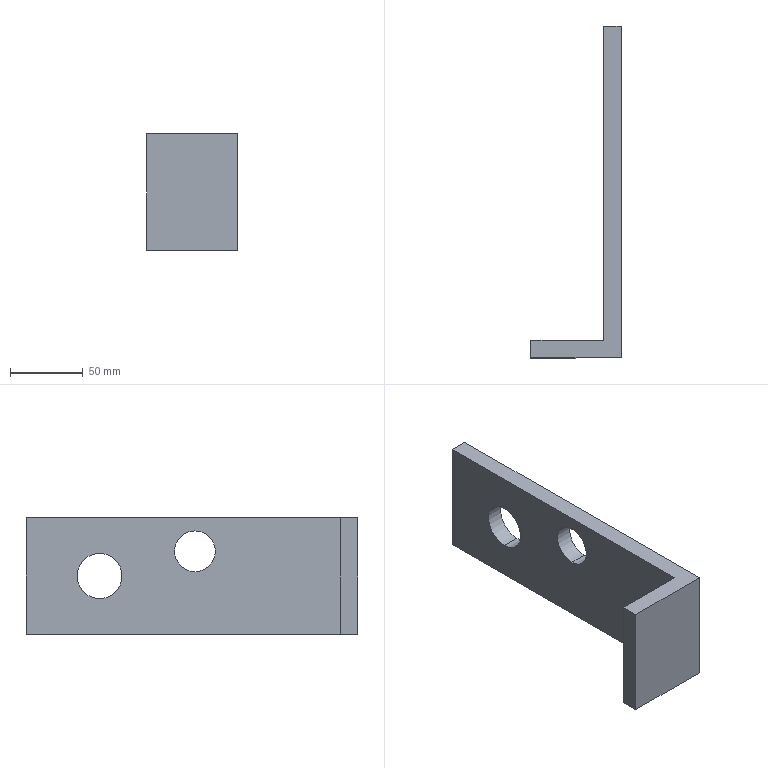Component | SolidWorks | HZ022-A001-E003-1 | 1 solid | 12 faces | box 62 x 228 x 80 mm | volume 250434 mm3 | plane 8 | cylinder 4 | commonest cylinder face diameters 28 x2 31 x2 | material AL6061
build123d program:
from build123d import *

# Parameters (mm, degrees)
SKETCH1_W           = 228
SKETCH1_H           = 80
BOSS_EXTRUDE1_DEPTH = 12
SKETCH2_W           = 80
SKETCH2_H           = 50
BOSS_EXTRUDE2_DEPTH = 12
CUT_EXTRUDE1_REACH  = 132.752
SKETCH5_R           = 15.5
SKETCH6_R           = 14
CUT_EXTRUDE2_DEPTH  = 131.752


with BuildPart() as part:
    # Sketch1 → Boss-Extrude1 (new body)
    with BuildSketch(Plane(origin=(0, 0, 0), x_dir=(1, 0, 0), z_dir=(0, 1, 0))):
        Rectangle(SKETCH1_W, SKETCH1_H)
    extrude(amount=BOSS_EXTRUDE1_DEPTH)

    # Sketch2 → Boss-Extrude2 (add)
    with BuildSketch(Plane.ZY.offset(114)):
        with Locations((0, 37)):
            Rectangle(SKETCH2_W, SKETCH2_H)
    extrude(amount=-BOSS_EXTRUDE2_DEPTH)

    # Sketch5 → Cut-Extrude1 (cut, up to next)
    with BuildSketch(Plane(origin=(0, 12, 0), x_dir=(1, 0, 0), z_dir=(0, 1, 0)), mode=Mode.PRIVATE) as cut_extrude1_sk1:
        with Locations(Location((63.5, 0, 0), (0, 0, 270))):
            Circle(SKETCH5_R)
    cut_extrude1_tool1 = extrude(cut_extrude1_sk1.sketch, amount=-CUT_EXTRUDE1_REACH, mode=Mode.PRIVATE) & part.part
    add(cut_extrude1_tool1.solids().sort_by_distance((63.5, 12, 0))[0], mode=Mode.SUBTRACT)

    # Sketch6 → Cut-Extrude2 (cut, through all)
    with BuildSketch(Plane(origin=(0, 12, 0), x_dir=(1, 0, 0), z_dir=(0, 1, 0))):
        with Locations(Location((-2, -17, 0), (0, 0, 270))):
            Circle(SKETCH6_R)
    extrude(amount=-CUT_EXTRUDE2_DEPTH, mode=Mode.SUBTRACT)


solid = part.part

# Placed as in the assembly
solid = solid.moved(Location((-77.556, 128.652, 910), (0, 0, 90)))
STEP:
#1=COLOUR_RGB('',0.7922,0.8196,0.9333);
#2=FILL_AREA_STYLE_COLOUR('',#1);
#3=FILL_AREA_STYLE('',(#2));
#4=SURFACE_STYLE_FILL_AREA(#3);
#5=SURFACE_SIDE_STYLE('',(#4));
#6=SURFACE_STYLE_USAGE(.BOTH.,#5);
#7=PRESENTATION_STYLE_ASSIGNMENT((#6));
#8=CARTESIAN_POINT('',(-3.053,4.986,35.945));
#9=VERTEX_POINT('',#8);
#10=CARTESIAN_POINT('',(-3.053,4.986,37.047));
#11=VERTEX_POINT('',#10);
#12=CARTESIAN_POINT('',(-3.053,4.986,36.496));
#13=DIRECTION('',(-1.,-0.,0.));
#14=DIRECTION('',(0.,0.,1.));
#15=AXIS2_PLACEMENT_3D('',#12,#13,#14);
#16=CIRCLE('',#15,0.5512);
#17=EDGE_CURVE('',#9,#11,#16,.T.);
#18=ORIENTED_EDGE('',*,*,#17,.F.);
#19=CARTESIAN_POINT('',(-3.526,4.986,35.945));
#20=VERTEX_POINT('',#19);
#21=CARTESIAN_POINT('',(-3.053,4.986,35.945));
#22=DIRECTION('',(-1.,-0.,0.));
#23=VECTOR('',#22,39.37);
#24=LINE('',#21,#23);
#25=EDGE_CURVE('',#9,#20,#24,.T.);
#26=ORIENTED_EDGE('',*,*,#25,.T.);
#27=CARTESIAN_POINT('',(-3.526,4.986,37.047));
#28=VERTEX_POINT('',#27);
#29=CARTESIAN_POINT('',(-3.526,4.986,36.496));
#30=DIRECTION('',(-1.,-0.,0.));
#31=DIRECTION('',(0.,0.,1.));
#32=AXIS2_PLACEMENT_3D('',#29,#30,#31);
#33=CIRCLE('',#32,0.5512);
#34=EDGE_CURVE('',#20,#28,#33,.T.);
#35=ORIENTED_EDGE('',*,*,#34,.T.);
#36=CARTESIAN_POINT('',(-3.053,4.986,37.047));
#37=DIRECTION('',(-1.,-0.,0.));
#38=VECTOR('',#37,39.37);
#39=LINE('',#36,#38);
#40=EDGE_CURVE('',#11,#28,#39,.T.);
#41=ORIENTED_EDGE('',*,*,#40,.F.);
#42=EDGE_LOOP('',(#18,#26,#35,#41));
#43=FACE_OUTER_BOUND('',#42,.T.);
#44=CARTESIAN_POINT('',(-3.053,4.986,36.496));
#45=DIRECTION('',(-1.,-0.,0.));
#46=DIRECTION('',(0.,0.,1.));
#47=AXIS2_PLACEMENT_3D('',#44,#45,#46);
#48=CYLINDRICAL_SURFACE('',#47,0.5512);
#49=ADVANCED_FACE('',(#43),#48,.F.);
#50=CARTESIAN_POINT('',(-3.053,7.565,36.437));
#51=VERTEX_POINT('',#50);
#52=CARTESIAN_POINT('',(-3.053,7.565,35.217));
#53=VERTEX_POINT('',#52);
#54=CARTESIAN_POINT('',(-3.053,7.565,35.827));
#55=DIRECTION('',(1.,0.,-0.));
#56=DIRECTION('',(0.,0.,1.));
#57=AXIS2_PLACEMENT_3D('',#54,#55,#56);
#58=CIRCLE('',#57,0.6102);
#59=EDGE_CURVE('',#51,#53,#58,.T.);
#60=ORIENTED_EDGE('',*,*,#59,.T.);
#61=CARTESIAN_POINT('',(-3.526,7.565,35.217));
#62=VERTEX_POINT('',#61);
#63=CARTESIAN_POINT('',(-3.053,7.565,35.217));
#64=DIRECTION('',(-1.,-0.,0.));
#65=VECTOR('',#64,39.37);
#66=LINE('',#63,#65);
#67=EDGE_CURVE('',#53,#62,#66,.T.);
#68=ORIENTED_EDGE('',*,*,#67,.T.);
#69=CARTESIAN_POINT('',(-3.526,7.565,36.437));
#70=VERTEX_POINT('',#69);
#71=CARTESIAN_POINT('',(-3.526,7.565,35.827));
#72=DIRECTION('',(-1.,-0.,0.));
#73=DIRECTION('',(0.,0.,1.));
#74=AXIS2_PLACEMENT_3D('',#71,#72,#73);
#75=CIRCLE('',#74,0.6102);
#76=EDGE_CURVE('',#62,#70,#75,.T.);
#77=ORIENTED_EDGE('',*,*,#76,.T.);
#78=CARTESIAN_POINT('',(-3.053,7.565,36.437));
#79=DIRECTION('',(-1.,-0.,0.));
#80=VECTOR('',#79,39.37);
#81=LINE('',#78,#80);
#82=EDGE_CURVE('',#51,#70,#81,.T.);
#83=ORIENTED_EDGE('',*,*,#82,.F.);
#84=EDGE_LOOP('',(#60,#68,#77,#83));
#85=FACE_OUTER_BOUND('',#84,.T.);
#86=CARTESIAN_POINT('',(-3.053,7.565,35.827));
#87=DIRECTION('',(-1.,-0.,0.));
#88=DIRECTION('',(0.,0.,1.));
#89=AXIS2_PLACEMENT_3D('',#86,#87,#88);
#90=CYLINDRICAL_SURFACE('',#89,0.6102);
#91=ADVANCED_FACE('',(#85),#90,.F.);
#92=CARTESIAN_POINT('',(-3.526,4.986,36.496));
#93=DIRECTION('',(-1.,-0.,0.));
#94=DIRECTION('',(0.,0.,1.));
#95=AXIS2_PLACEMENT_3D('',#92,#93,#94);
#96=CIRCLE('',#95,0.5512);
#97=EDGE_CURVE('',#28,#20,#96,.T.);
#98=ORIENTED_EDGE('',*,*,#97,.F.);
#99=ORIENTED_EDGE('',*,*,#34,.F.);
#100=EDGE_LOOP('',(#98,#99));
#101=FACE_BOUND('',#100,.T.);
#102=CARTESIAN_POINT('',(-3.526,7.565,35.827));
#103=DIRECTION('',(-1.,-0.,0.));
#104=DIRECTION('',(0.,0.,1.));
#105=AXIS2_PLACEMENT_3D('',#102,#103,#104);
#106=CIRCLE('',#105,0.6102);
#107=EDGE_CURVE('',#70,#62,#106,.T.);
#108=ORIENTED_EDGE('',*,*,#107,.F.);
#109=ORIENTED_EDGE('',*,*,#76,.F.);
#110=EDGE_LOOP('',(#108,#109));
#111=FACE_BOUND('',#110,.T.);
#112=CARTESIAN_POINT('',(-3.526,9.553,34.252));
#113=VERTEX_POINT('',#112);
#114=CARTESIAN_POINT('',(-3.526,1.049,34.252));
#115=VERTEX_POINT('',#114);
#116=CARTESIAN_POINT('',(-3.526,0.5769,34.252));
#117=DIRECTION('',(0.,-1.,-0.));
#118=VECTOR('',#117,39.37);
#119=LINE('',#116,#118);
#120=EDGE_CURVE('',#113,#115,#119,.T.);
#121=ORIENTED_EDGE('',*,*,#120,.T.);
#122=CARTESIAN_POINT('',(-3.526,1.049,37.402));
#123=VERTEX_POINT('',#122);
#124=CARTESIAN_POINT('',(-3.526,1.049,34.252));
#125=DIRECTION('',(0.,0.,1.));
#126=VECTOR('',#125,39.37);
#127=LINE('',#124,#126);
#128=EDGE_CURVE('',#115,#123,#127,.T.);
#129=ORIENTED_EDGE('',*,*,#128,.T.);
#130=CARTESIAN_POINT('',(-3.526,9.553,37.402));
#131=VERTEX_POINT('',#130);
#132=CARTESIAN_POINT('',(-3.526,0.5769,37.402));
#133=DIRECTION('',(-0.,1.,0.));
#134=VECTOR('',#133,39.37);
#135=LINE('',#132,#134);
#136=EDGE_CURVE('',#123,#131,#135,.T.);
#137=ORIENTED_EDGE('',*,*,#136,.T.);
#138=CARTESIAN_POINT('',(-3.526,9.553,34.252));
#139=DIRECTION('',(-0.,-0.,-1.));
#140=VECTOR('',#139,39.37);
#141=LINE('',#138,#140);
#142=EDGE_CURVE('',#131,#113,#141,.T.);
#143=ORIENTED_EDGE('',*,*,#142,.T.);
#144=EDGE_LOOP('',(#121,#129,#137,#143));
#145=FACE_OUTER_BOUND('',#144,.T.);
#146=CARTESIAN_POINT('',(-3.526,5.065,35.827));
#147=DIRECTION('',(-1.,-0.,0.));
#148=DIRECTION('',(0.,-0.,1.));
#149=AXIS2_PLACEMENT_3D('',#146,#147,#148);
#150=PLANE('',#149);
#151=ADVANCED_FACE('',(#101,#111,#145),#150,.T.);
#152=CARTESIAN_POINT('',(-3.053,9.553,37.402));
#153=VERTEX_POINT('',#152);
#154=CARTESIAN_POINT('',(-3.053,9.553,34.252));
#155=VERTEX_POINT('',#154);
#156=CARTESIAN_POINT('',(-3.053,9.553,34.252));
#157=DIRECTION('',(-0.,-0.,-1.));
#158=VECTOR('',#157,39.37);
#159=LINE('',#156,#158);
#160=EDGE_CURVE('',#153,#155,#159,.T.);
#161=ORIENTED_EDGE('',*,*,#160,.T.);
#162=CARTESIAN_POINT('',(-3.526,9.553,34.252));
#163=DIRECTION('',(1.,0.,-0.));
#164=VECTOR('',#163,39.37);
#165=LINE('',#162,#164);
#166=EDGE_CURVE('',#113,#155,#165,.T.);
#167=ORIENTED_EDGE('',*,*,#166,.F.);
#168=ORIENTED_EDGE('',*,*,#142,.F.);
#169=CARTESIAN_POINT('',(-3.526,9.553,37.402));
#170=DIRECTION('',(1.,0.,-0.));
#171=VECTOR('',#170,39.37);
#172=LINE('',#169,#171);
#173=EDGE_CURVE('',#131,#153,#172,.T.);
#174=ORIENTED_EDGE('',*,*,#173,.T.);
#175=EDGE_LOOP('',(#161,#167,#168,#174));
#176=FACE_OUTER_BOUND('',#175,.T.);
#177=CARTESIAN_POINT('',(-3.526,9.553,34.252));
#178=DIRECTION('',(0.,-1.,0.));
#179=DIRECTION('',(0.,0.,1.));
#180=AXIS2_PLACEMENT_3D('',#177,#178,#179);
#181=PLANE('',#180);
#182=ADVANCED_FACE('',(#176),#181,.F.);
#183=CARTESIAN_POINT('',(-3.053,0.5769,34.252));
#184=VERTEX_POINT('',#183);
#185=CARTESIAN_POINT('',(-3.053,0.5769,34.252));
#186=DIRECTION('',(0.,-1.,-0.));
#187=VECTOR('',#186,39.37);
#188=LINE('',#185,#187);
#189=EDGE_CURVE('',#155,#184,#188,.T.);
#190=ORIENTED_EDGE('',*,*,#189,.T.);
#191=CARTESIAN_POINT('',(-5.494,0.5769,34.252));
#192=VERTEX_POINT('',#191);
#193=CARTESIAN_POINT('',(-3.526,0.5769,34.252));
#194=DIRECTION('',(1.,0.,-0.));
#195=VECTOR('',#194,39.37);
#196=LINE('',#193,#195);
#197=EDGE_CURVE('',#192,#184,#196,.T.);
#198=ORIENTED_EDGE('',*,*,#197,.F.);
#199=CARTESIAN_POINT('',(-5.494,1.049,34.252));
#200=VERTEX_POINT('',#199);
#201=CARTESIAN_POINT('',(-5.494,1.049,34.252));
#202=DIRECTION('',(0.,-1.,0.));
#203=VECTOR('',#202,39.37);
#204=LINE('',#201,#203);
#205=EDGE_CURVE('',#200,#192,#204,.T.);
#206=ORIENTED_EDGE('',*,*,#205,.F.);
#207=CARTESIAN_POINT('',(-3.526,1.049,34.252));
#208=DIRECTION('',(1.,0.,-0.));
#209=VECTOR('',#208,39.37);
#210=LINE('',#207,#209);
#211=EDGE_CURVE('',#200,#115,#210,.T.);
#212=ORIENTED_EDGE('',*,*,#211,.T.);
#213=ORIENTED_EDGE('',*,*,#120,.F.);
#214=ORIENTED_EDGE('',*,*,#166,.T.);
#215=EDGE_LOOP('',(#190,#198,#206,#212,#213,#214));
#216=FACE_OUTER_BOUND('',#215,.T.);
#217=CARTESIAN_POINT('',(-3.526,0.5769,34.252));
#218=DIRECTION('',(0.,-0.,1.));
#219=DIRECTION('',(-0.,1.,0.));
#220=AXIS2_PLACEMENT_3D('',#217,#218,#219);
#221=PLANE('',#220);
#222=ADVANCED_FACE('',(#216),#221,.F.);
#223=CARTESIAN_POINT('',(-3.053,0.5769,37.402));
#224=VERTEX_POINT('',#223);
#225=CARTESIAN_POINT('',(-3.053,0.5769,34.252));
#226=DIRECTION('',(0.,-0.,1.));
#227=VECTOR('',#226,39.37);
#228=LINE('',#225,#227);
#229=EDGE_CURVE('',#184,#224,#228,.T.);
#230=ORIENTED_EDGE('',*,*,#229,.T.);
#231=CARTESIAN_POINT('',(-5.494,0.5769,37.402));
#232=VERTEX_POINT('',#231);
#233=CARTESIAN_POINT('',(-3.526,0.5769,37.402));
#234=DIRECTION('',(1.,0.,-0.));
#235=VECTOR('',#234,39.37);
#236=LINE('',#233,#235);
#237=EDGE_CURVE('',#232,#224,#236,.T.);
#238=ORIENTED_EDGE('',*,*,#237,.F.);
#239=CARTESIAN_POINT('',(-5.494,0.5769,34.252));
#240=DIRECTION('',(-0.,-0.,-1.));
#241=VECTOR('',#240,39.37);
#242=LINE('',#239,#241);
#243=EDGE_CURVE('',#232,#192,#242,.T.);
#244=ORIENTED_EDGE('',*,*,#243,.T.);
#245=ORIENTED_EDGE('',*,*,#197,.T.);
#246=EDGE_LOOP('',(#230,#238,#244,#245));
#247=FACE_OUTER_BOUND('',#246,.T.);
#248=CARTESIAN_POINT('',(-3.526,0.5769,34.252));
#249=DIRECTION('',(-0.,1.,0.));
#250=DIRECTION('',(-0.,0.,-1.));
#251=AXIS2_PLACEMENT_3D('',#248,#249,#250);
#252=PLANE('',#251);
#253=ADVANCED_FACE('',(#247),#252,.F.);
#254=CARTESIAN_POINT('',(-3.053,0.5769,37.402));
#255=DIRECTION('',(-0.,1.,0.));
#256=VECTOR('',#255,39.37);
#257=LINE('',#254,#256);
#258=EDGE_CURVE('',#224,#153,#257,.T.);
#259=ORIENTED_EDGE('',*,*,#258,.T.);
#260=ORIENTED_EDGE('',*,*,#173,.F.);
#261=ORIENTED_EDGE('',*,*,#136,.F.);
#262=CARTESIAN_POINT('',(-5.494,1.049,37.402));
#263=VERTEX_POINT('',#262);
#264=CARTESIAN_POINT('',(-3.526,1.049,37.402));
#265=DIRECTION('',(-1.,-0.,0.));
#266=VECTOR('',#265,39.37);
#267=LINE('',#264,#266);
#268=EDGE_CURVE('',#123,#263,#267,.T.);
#269=ORIENTED_EDGE('',*,*,#268,.T.);
#270=CARTESIAN_POINT('',(-5.494,1.049,37.402));
#271=DIRECTION('',(0.,-1.,0.));
#272=VECTOR('',#271,39.37);
#273=LINE('',#270,#272);
#274=EDGE_CURVE('',#263,#232,#273,.T.);
#275=ORIENTED_EDGE('',*,*,#274,.T.);
#276=ORIENTED_EDGE('',*,*,#237,.T.);
#277=EDGE_LOOP('',(#259,#260,#261,#269,#275,#276));
#278=FACE_OUTER_BOUND('',#277,.T.);
#279=CARTESIAN_POINT('',(-3.526,0.5769,37.402));
#280=DIRECTION('',(-0.,0.,-1.));
#281=DIRECTION('',(0.,-1.,-0.));
#282=AXIS2_PLACEMENT_3D('',#279,#280,#281);
#283=PLANE('',#282);
#284=ADVANCED_FACE('',(#278),#283,.F.);
#285=CARTESIAN_POINT('',(-3.053,4.986,36.496));
#286=DIRECTION('',(-1.,-0.,0.));
#287=DIRECTION('',(0.,0.,1.));
#288=AXIS2_PLACEMENT_3D('',#285,#286,#287);
#289=CIRCLE('',#288,0.5512);
#290=EDGE_CURVE('',#11,#9,#289,.T.);
#291=ORIENTED_EDGE('',*,*,#290,.T.);
#292=ORIENTED_EDGE('',*,*,#17,.T.);
#293=EDGE_LOOP('',(#291,#292));
#294=FACE_BOUND('',#293,.T.);
#295=ORIENTED_EDGE('',*,*,#59,.F.);
#296=CARTESIAN_POINT('',(-3.053,7.565,35.827));
#297=DIRECTION('',(1.,0.,-0.));
#298=DIRECTION('',(0.,0.,1.));
#299=AXIS2_PLACEMENT_3D('',#296,#297,#298);
#300=CIRCLE('',#299,0.6102);
#301=EDGE_CURVE('',#53,#51,#300,.T.);
#302=ORIENTED_EDGE('',*,*,#301,.F.);
#303=EDGE_LOOP('',(#295,#302));
#304=FACE_BOUND('',#303,.T.);
#305=ORIENTED_EDGE('',*,*,#160,.F.);
#306=ORIENTED_EDGE('',*,*,#258,.F.);
#307=ORIENTED_EDGE('',*,*,#229,.F.);
#308=ORIENTED_EDGE('',*,*,#189,.F.);
#309=EDGE_LOOP('',(#305,#306,#307,#308));
#310=FACE_OUTER_BOUND('',#309,.T.);
#311=CARTESIAN_POINT('',(-3.053,5.065,35.827));
#312=DIRECTION('',(-1.,-0.,0.));
#313=DIRECTION('',(0.,-0.,1.));
#314=AXIS2_PLACEMENT_3D('',#311,#312,#313);
#315=PLANE('',#314);
#316=ADVANCED_FACE('',(#294,#304,#310),#315,.F.);
#317=ORIENTED_EDGE('',*,*,#243,.F.);
#318=ORIENTED_EDGE('',*,*,#274,.F.);
#319=CARTESIAN_POINT('',(-5.494,1.049,34.252));
#320=DIRECTION('',(-0.,-0.,-1.));
#321=VECTOR('',#320,39.37);
#322=LINE('',#319,#321);
#323=EDGE_CURVE('',#263,#200,#322,.T.);
#324=ORIENTED_EDGE('',*,*,#323,.T.);
#325=ORIENTED_EDGE('',*,*,#205,.T.);
#326=EDGE_LOOP('',(#317,#318,#324,#325));
#327=FACE_OUTER_BOUND('',#326,.T.);
#328=CARTESIAN_POINT('',(-5.494,1.049,34.252));
#329=DIRECTION('',(-1.,-0.,0.));
#330=DIRECTION('',(0.,-0.,1.));
#331=AXIS2_PLACEMENT_3D('',#328,#329,#330);
#332=PLANE('',#331);
#333=ADVANCED_FACE('',(#327),#332,.T.);
#334=ORIENTED_EDGE('',*,*,#211,.F.);
#335=ORIENTED_EDGE('',*,*,#323,.F.);
#336=ORIENTED_EDGE('',*,*,#268,.F.);
#337=ORIENTED_EDGE('',*,*,#128,.F.);
#338=EDGE_LOOP('',(#334,#335,#336,#337));
#339=FACE_OUTER_BOUND('',#338,.T.);
#340=CARTESIAN_POINT('',(-3.053,1.049,35.827));
#341=DIRECTION('',(-0.,1.,-0.));
#342=DIRECTION('',(-0.,-0.,-1.));
#343=AXIS2_PLACEMENT_3D('',#340,#341,#342);
#344=PLANE('',#343);
#345=ADVANCED_FACE('',(#339),#344,.T.);
#346=ORIENTED_EDGE('',*,*,#67,.F.);
#347=ORIENTED_EDGE('',*,*,#301,.T.);
#348=ORIENTED_EDGE('',*,*,#82,.T.);
#349=ORIENTED_EDGE('',*,*,#107,.T.);
#350=EDGE_LOOP('',(#346,#347,#348,#349));
#351=FACE_OUTER_BOUND('',#350,.T.);
#352=CARTESIAN_POINT('',(-3.053,7.565,35.827));
#353=DIRECTION('',(-1.,-0.,0.));
#354=DIRECTION('',(0.,0.,1.));
#355=AXIS2_PLACEMENT_3D('',#352,#353,#354);
#356=CYLINDRICAL_SURFACE('',#355,0.6102);
#357=ADVANCED_FACE('',(#351),#356,.F.);
#358=ORIENTED_EDGE('',*,*,#25,.F.);
#359=ORIENTED_EDGE('',*,*,#290,.F.);
#360=ORIENTED_EDGE('',*,*,#40,.T.);
#361=ORIENTED_EDGE('',*,*,#97,.T.);
#362=EDGE_LOOP('',(#358,#359,#360,#361));
#363=FACE_OUTER_BOUND('',#362,.T.);
#364=CARTESIAN_POINT('',(-3.053,4.986,36.496));
#365=DIRECTION('',(-1.,-0.,0.));
#366=DIRECTION('',(0.,0.,1.));
#367=AXIS2_PLACEMENT_3D('',#364,#365,#366);
#368=CYLINDRICAL_SURFACE('',#367,0.5512);
#369=ADVANCED_FACE('',(#363),#368,.F.);
#370=CLOSED_SHELL('',(#49,#91,#151,#182,#222,#253,#284,#316,#333,#345,#357,#369));
#371=MANIFOLD_SOLID_BREP('',#370);
#372=STYLED_ITEM('',(#7),#371);
#373=PRESENTATION_LAYER_ASSIGNMENT('','',(#372));
#374=(LENGTH_UNIT()NAMED_UNIT(*)SI_UNIT($,.METRE.));
#375=LENGTH_MEASURE_WITH_UNIT(LENGTH_MEASURE(0.0254),#374);
#376=DIMENSIONAL_EXPONENTS(1.,0.,0.,0.,0.,0.,0.);
#377=(CONVERSION_BASED_UNIT('',#375)LENGTH_UNIT()NAMED_UNIT(#376));
#378=UNCERTAINTY_MEASURE_WITH_UNIT(LENGTH_MEASURE(0.00001),#377,'','');
#379=(NAMED_UNIT(*)PLANE_ANGLE_UNIT()SI_UNIT($,.RADIAN.));
#380=(NAMED_UNIT(*)SI_UNIT($,.STERADIAN.)SOLID_ANGLE_UNIT());
#381=(GEOMETRIC_REPRESENTATION_CONTEXT(3)GLOBAL_UNCERTAINTY_ASSIGNED_CONTEXT((#378))GLOBAL_UNIT_ASSIGNED_CONTEXT((#377,#379,#380))REPRESENTATION_CONTEXT('',''));
#382=MECHANICAL_DESIGN_GEOMETRIC_PRESENTATION_REPRESENTATION('',(#372),#381);
#383=CARTESIAN_POINT('',(0.,0.,0.));
#384=DIRECTION('',(0.,0.,1.));
#385=DIRECTION('',(1.,0.,0.));
#386=AXIS2_PLACEMENT_3D('',#383,#384,#385);
#387=(LENGTH_UNIT()NAMED_UNIT(*)SI_UNIT($,.METRE.));
#388=LENGTH_MEASURE_WITH_UNIT(LENGTH_MEASURE(0.0254),#387);
#389=DIMENSIONAL_EXPONENTS(1.,0.,0.,0.,0.,0.,0.);
#390=(CONVERSION_BASED_UNIT('',#388)LENGTH_UNIT()NAMED_UNIT(#389));
#391=UNCERTAINTY_MEASURE_WITH_UNIT(LENGTH_MEASURE(0.00001),#390,'','');
#392=(NAMED_UNIT(*)PLANE_ANGLE_UNIT()SI_UNIT($,.RADIAN.));
#393=(NAMED_UNIT(*)SI_UNIT($,.STERADIAN.)SOLID_ANGLE_UNIT());
#394=(GEOMETRIC_REPRESENTATION_CONTEXT(3)GLOBAL_UNCERTAINTY_ASSIGNED_CONTEXT((#391))GLOBAL_UNIT_ASSIGNED_CONTEXT((#390,#392,#393))REPRESENTATION_CONTEXT('',''));
#395=ADVANCED_BREP_SHAPE_REPRESENTATION('',(#371,#386),#394);